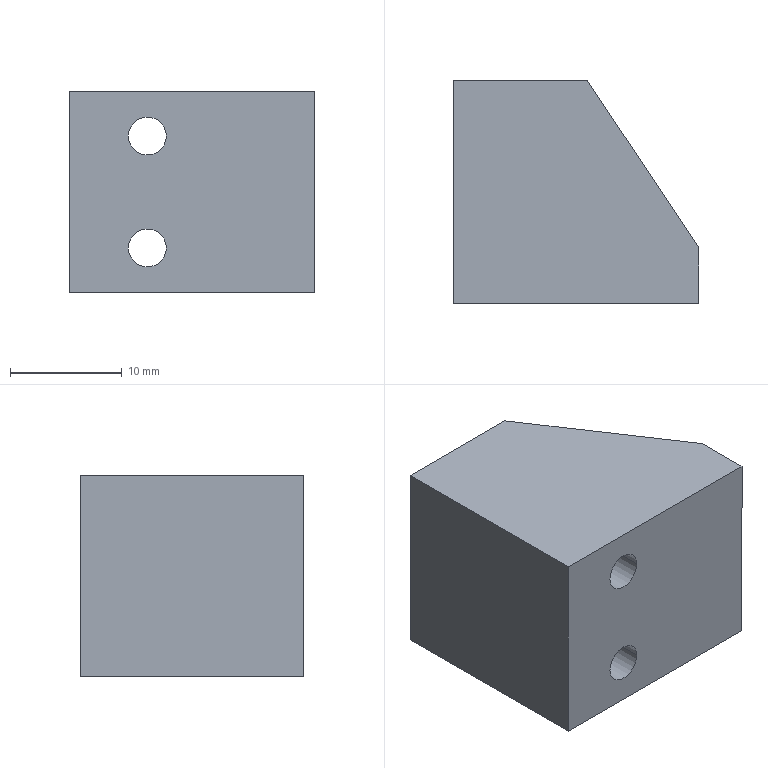Component | SolidWorks | XM-02-008A1-1 | 1 solid | 17 faces | box 22 x 20 x 18 mm | volume 5823 mm3 | plane 9 | cylinder 8 | commonest cylinder face diameters 6 x4 3.4 x4 | material Black POM
build123d program:
from build123d import *

# Parameters (mm, degrees)
SKETCH1_W                                          = 18
SKETCH1_H                                          = 22
BOSS_EXTRUDE1_DEPTH                                = 20
CUT_EXTRUDE1_DEPTH                                 = 20
HOLE_SIZE_ACCORDING_TO_TYPE_1_OF_HEX_S_D           = 3.4
HOLE_SIZE_ACCORDING_TO_TYPE_1_OF_HEX_S_CBORE_D     = 6
HOLE_SIZE_ACCORDING_TO_TYPE_1_OF_HEX_S_CBORE_DEPTH = 10


with BuildPart() as part:
    # Sketch1 → Boss-Extrude1 (new body)
    with BuildSketch(Plane(origin=(0, 0, 0), x_dir=(1, 0, 0), z_dir=(0, 1, 0))):
        Rectangle(SKETCH1_W, SKETCH1_H)
    extrude(amount=BOSS_EXTRUDE1_DEPTH)

    # Sketch14 → Cut-Extrude1 (cut)
    with BuildSketch(Plane.ZY.offset(9)):
        Polygon((-11, 20), (-1, 20), (-11, 5), align=None)
    extrude(amount=-CUT_EXTRUDE1_DEPTH, mode=Mode.SUBTRACT)

    # Hole Size _according to_ Type 1 of Hex S (through all)
    with Locations(Plane(origin=(0, 20, 0), x_dir=(1, 0, 0), z_dir=(0, 1, 0))):
        with Locations((5, -4), (-5, -4)):
            CounterBoreHole(HOLE_SIZE_ACCORDING_TO_TYPE_1_OF_HEX_S_D / 2, HOLE_SIZE_ACCORDING_TO_TYPE_1_OF_HEX_S_CBORE_D / 2, HOLE_SIZE_ACCORDING_TO_TYPE_1_OF_HEX_S_CBORE_DEPTH)


solid = part.part

# Placed as in the assembly
solid = solid.moved(Location((-54, 0, 0), (0, -90, 0)))
STEP:
#1=COLOUR_RGB('',0.7922,0.8196,0.9333);
#2=FILL_AREA_STYLE_COLOUR('',#1);
#3=FILL_AREA_STYLE('',(#2));
#4=SURFACE_STYLE_FILL_AREA(#3);
#5=SURFACE_SIDE_STYLE('',(#4));
#6=SURFACE_STYLE_USAGE(.BOTH.,#5);
#7=PRESENTATION_STYLE_ASSIGNMENT((#6));
#8=CARTESIAN_POINT('',(-2.165,0.3937,0.1969));
#9=VERTEX_POINT('',#8);
#10=CARTESIAN_POINT('',(-2.402,0.3937,0.1969));
#11=VERTEX_POINT('',#10);
#12=CARTESIAN_POINT('',(-2.283,0.3937,0.1969));
#13=DIRECTION('',(0.,1.,-0.));
#14=DIRECTION('',(-1.,0.,0.));
#15=AXIS2_PLACEMENT_3D('',#12,#13,#14);
#16=CIRCLE('',#15,0.1181);
#17=EDGE_CURVE('',#9,#11,#16,.T.);
#18=ORIENTED_EDGE('',*,*,#17,.F.);
#19=CARTESIAN_POINT('',(-2.165,0.7874,0.1969));
#20=VERTEX_POINT('',#19);
#21=CARTESIAN_POINT('',(-2.165,0.7874,0.1969));
#22=DIRECTION('',(0.,1.,-0.));
#23=VECTOR('',#22,39.37);
#24=LINE('',#21,#23);
#25=EDGE_CURVE('',#9,#20,#24,.T.);
#26=ORIENTED_EDGE('',*,*,#25,.T.);
#27=CARTESIAN_POINT('',(-2.402,0.7874,0.1969));
#28=VERTEX_POINT('',#27);
#29=CARTESIAN_POINT('',(-2.283,0.7874,0.1969));
#30=DIRECTION('',(0.,1.,-0.));
#31=DIRECTION('',(-1.,0.,0.));
#32=AXIS2_PLACEMENT_3D('',#29,#30,#31);
#33=CIRCLE('',#32,0.1181);
#34=EDGE_CURVE('',#20,#28,#33,.T.);
#35=ORIENTED_EDGE('',*,*,#34,.T.);
#36=CARTESIAN_POINT('',(-2.402,0.7874,0.1969));
#37=DIRECTION('',(0.,1.,-0.));
#38=VECTOR('',#37,39.37);
#39=LINE('',#36,#38);
#40=EDGE_CURVE('',#11,#28,#39,.T.);
#41=ORIENTED_EDGE('',*,*,#40,.F.);
#42=EDGE_LOOP('',(#18,#26,#35,#41));
#43=FACE_OUTER_BOUND('',#42,.T.);
#44=CARTESIAN_POINT('',(-2.283,0.7874,0.1969));
#45=DIRECTION('',(0.,1.,-0.));
#46=DIRECTION('',(-1.,0.,0.));
#47=AXIS2_PLACEMENT_3D('',#44,#45,#46);
#48=CYLINDRICAL_SURFACE('',#47,0.1181);
#49=ADVANCED_FACE('',(#43),#48,.F.);
#50=CARTESIAN_POINT('',(-2.217,0.,0.1969));
#51=VERTEX_POINT('',#50);
#52=CARTESIAN_POINT('',(-2.35,0.,0.1969));
#53=VERTEX_POINT('',#52);
#54=CARTESIAN_POINT('',(-2.283,0.,0.1969));
#55=DIRECTION('',(0.,1.,-0.));
#56=DIRECTION('',(-1.,0.,0.));
#57=AXIS2_PLACEMENT_3D('',#54,#55,#56);
#58=CIRCLE('',#57,0.06693);
#59=EDGE_CURVE('',#51,#53,#58,.T.);
#60=ORIENTED_EDGE('',*,*,#59,.F.);
#61=CARTESIAN_POINT('',(-2.217,0.3937,0.1969));
#62=VERTEX_POINT('',#61);
#63=CARTESIAN_POINT('',(-2.217,0.7874,0.1969));
#64=DIRECTION('',(0.,1.,-0.));
#65=VECTOR('',#64,39.37);
#66=LINE('',#63,#65);
#67=EDGE_CURVE('',#51,#62,#66,.T.);
#68=ORIENTED_EDGE('',*,*,#67,.T.);
#69=CARTESIAN_POINT('',(-2.35,0.3937,0.1969));
#70=VERTEX_POINT('',#69);
#71=CARTESIAN_POINT('',(-2.283,0.3937,0.1969));
#72=DIRECTION('',(0.,1.,-0.));
#73=DIRECTION('',(-1.,0.,0.));
#74=AXIS2_PLACEMENT_3D('',#71,#72,#73);
#75=CIRCLE('',#74,0.06693);
#76=EDGE_CURVE('',#62,#70,#75,.T.);
#77=ORIENTED_EDGE('',*,*,#76,.T.);
#78=CARTESIAN_POINT('',(-2.35,0.7874,0.1969));
#79=DIRECTION('',(0.,1.,-0.));
#80=VECTOR('',#79,39.37);
#81=LINE('',#78,#80);
#82=EDGE_CURVE('',#53,#70,#81,.T.);
#83=ORIENTED_EDGE('',*,*,#82,.F.);
#84=EDGE_LOOP('',(#60,#68,#77,#83));
#85=FACE_OUTER_BOUND('',#84,.T.);
#86=CARTESIAN_POINT('',(-2.283,0.7874,0.1969));
#87=DIRECTION('',(0.,1.,-0.));
#88=DIRECTION('',(-1.,0.,0.));
#89=AXIS2_PLACEMENT_3D('',#86,#87,#88);
#90=CYLINDRICAL_SURFACE('',#89,0.06693);
#91=ADVANCED_FACE('',(#85),#90,.F.);
#92=CARTESIAN_POINT('',(-2.165,0.3937,-0.1969));
#93=VERTEX_POINT('',#92);
#94=CARTESIAN_POINT('',(-2.402,0.3937,-0.1969));
#95=VERTEX_POINT('',#94);
#96=CARTESIAN_POINT('',(-2.283,0.3937,-0.1969));
#97=DIRECTION('',(0.,1.,-0.));
#98=DIRECTION('',(-1.,0.,0.));
#99=AXIS2_PLACEMENT_3D('',#96,#97,#98);
#100=CIRCLE('',#99,0.1181);
#101=EDGE_CURVE('',#93,#95,#100,.T.);
#102=ORIENTED_EDGE('',*,*,#101,.F.);
#103=CARTESIAN_POINT('',(-2.165,0.7874,-0.1969));
#104=VERTEX_POINT('',#103);
#105=CARTESIAN_POINT('',(-2.165,0.7874,-0.1969));
#106=DIRECTION('',(0.,1.,-0.));
#107=VECTOR('',#106,39.37);
#108=LINE('',#105,#107);
#109=EDGE_CURVE('',#93,#104,#108,.T.);
#110=ORIENTED_EDGE('',*,*,#109,.T.);
#111=CARTESIAN_POINT('',(-2.402,0.7874,-0.1969));
#112=VERTEX_POINT('',#111);
#113=CARTESIAN_POINT('',(-2.283,0.7874,-0.1969));
#114=DIRECTION('',(0.,1.,-0.));
#115=DIRECTION('',(-1.,0.,0.));
#116=AXIS2_PLACEMENT_3D('',#113,#114,#115);
#117=CIRCLE('',#116,0.1181);
#118=EDGE_CURVE('',#104,#112,#117,.T.);
#119=ORIENTED_EDGE('',*,*,#118,.T.);
#120=CARTESIAN_POINT('',(-2.402,0.7874,-0.1969));
#121=DIRECTION('',(0.,1.,-0.));
#122=VECTOR('',#121,39.37);
#123=LINE('',#120,#122);
#124=EDGE_CURVE('',#95,#112,#123,.T.);
#125=ORIENTED_EDGE('',*,*,#124,.F.);
#126=EDGE_LOOP('',(#102,#110,#119,#125));
#127=FACE_OUTER_BOUND('',#126,.T.);
#128=CARTESIAN_POINT('',(-2.283,0.7874,-0.1969));
#129=DIRECTION('',(0.,1.,-0.));
#130=DIRECTION('',(-1.,0.,0.));
#131=AXIS2_PLACEMENT_3D('',#128,#129,#130);
#132=CYLINDRICAL_SURFACE('',#131,0.1181);
#133=ADVANCED_FACE('',(#127),#132,.F.);
#134=CARTESIAN_POINT('',(-2.217,0.,-0.1969));
#135=VERTEX_POINT('',#134);
#136=CARTESIAN_POINT('',(-2.35,0.,-0.1969));
#137=VERTEX_POINT('',#136);
#138=CARTESIAN_POINT('',(-2.283,0.,-0.1969));
#139=DIRECTION('',(0.,1.,-0.));
#140=DIRECTION('',(-1.,0.,0.));
#141=AXIS2_PLACEMENT_3D('',#138,#139,#140);
#142=CIRCLE('',#141,0.06693);
#143=EDGE_CURVE('',#135,#137,#142,.T.);
#144=ORIENTED_EDGE('',*,*,#143,.F.);
#145=CARTESIAN_POINT('',(-2.217,0.3937,-0.1969));
#146=VERTEX_POINT('',#145);
#147=CARTESIAN_POINT('',(-2.217,0.7874,-0.1969));
#148=DIRECTION('',(0.,1.,-0.));
#149=VECTOR('',#148,39.37);
#150=LINE('',#147,#149);
#151=EDGE_CURVE('',#135,#146,#150,.T.);
#152=ORIENTED_EDGE('',*,*,#151,.T.);
#153=CARTESIAN_POINT('',(-2.35,0.3937,-0.1969));
#154=VERTEX_POINT('',#153);
#155=CARTESIAN_POINT('',(-2.283,0.3937,-0.1969));
#156=DIRECTION('',(0.,1.,-0.));
#157=DIRECTION('',(-1.,0.,0.));
#158=AXIS2_PLACEMENT_3D('',#155,#156,#157);
#159=CIRCLE('',#158,0.06693);
#160=EDGE_CURVE('',#146,#154,#159,.T.);
#161=ORIENTED_EDGE('',*,*,#160,.T.);
#162=CARTESIAN_POINT('',(-2.35,0.7874,-0.1969));
#163=DIRECTION('',(0.,1.,-0.));
#164=VECTOR('',#163,39.37);
#165=LINE('',#162,#164);
#166=EDGE_CURVE('',#137,#154,#165,.T.);
#167=ORIENTED_EDGE('',*,*,#166,.F.);
#168=EDGE_LOOP('',(#144,#152,#161,#167));
#169=FACE_OUTER_BOUND('',#168,.T.);
#170=CARTESIAN_POINT('',(-2.283,0.7874,-0.1969));
#171=DIRECTION('',(0.,1.,-0.));
#172=DIRECTION('',(-1.,0.,0.));
#173=AXIS2_PLACEMENT_3D('',#170,#171,#172);
#174=CYLINDRICAL_SURFACE('',#173,0.06693);
#175=ADVANCED_FACE('',(#169),#174,.F.);
#176=CARTESIAN_POINT('',(-1.693,0.1969,0.3543));
#177=VERTEX_POINT('',#176);
#178=CARTESIAN_POINT('',(-1.693,0.,0.3543));
#179=VERTEX_POINT('',#178);
#180=CARTESIAN_POINT('',(-1.693,0.7874,0.3543));
#181=DIRECTION('',(-0.,-1.,0.));
#182=VECTOR('',#181,39.37);
#183=LINE('',#180,#182);
#184=EDGE_CURVE('',#177,#179,#183,.T.);
#185=ORIENTED_EDGE('',*,*,#184,.F.);
#186=CARTESIAN_POINT('',(-2.087,0.7874,0.3543));
#187=VERTEX_POINT('',#186);
#188=CARTESIAN_POINT('',(-1.965,0.6057,0.3543));
#189=DIRECTION('',(-0.5547,0.8321,0.));
#190=VECTOR('',#189,39.37);
#191=LINE('',#188,#190);
#192=EDGE_CURVE('',#177,#187,#191,.T.);
#193=ORIENTED_EDGE('',*,*,#192,.T.);
#194=CARTESIAN_POINT('',(-2.559,0.7874,0.3543));
#195=VERTEX_POINT('',#194);
#196=CARTESIAN_POINT('',(-1.693,0.7874,0.3543));
#197=DIRECTION('',(1.,-0.,-0.));
#198=VECTOR('',#197,39.37);
#199=LINE('',#196,#198);
#200=EDGE_CURVE('',#195,#187,#199,.T.);
#201=ORIENTED_EDGE('',*,*,#200,.F.);
#202=CARTESIAN_POINT('',(-2.559,0.,0.3543));
#203=VERTEX_POINT('',#202);
#204=CARTESIAN_POINT('',(-2.559,0.7874,0.3543));
#205=DIRECTION('',(-0.,-1.,0.));
#206=VECTOR('',#205,39.37);
#207=LINE('',#204,#206);
#208=EDGE_CURVE('',#195,#203,#207,.T.);
#209=ORIENTED_EDGE('',*,*,#208,.T.);
#210=CARTESIAN_POINT('',(-1.693,0.,0.3543));
#211=DIRECTION('',(1.,-0.,-0.));
#212=VECTOR('',#211,39.37);
#213=LINE('',#210,#212);
#214=EDGE_CURVE('',#203,#179,#213,.T.);
#215=ORIENTED_EDGE('',*,*,#214,.T.);
#216=EDGE_LOOP('',(#185,#193,#201,#209,#215));
#217=FACE_OUTER_BOUND('',#216,.T.);
#218=CARTESIAN_POINT('',(-1.693,0.7874,0.3543));
#219=DIRECTION('',(-0.,-0.,-1.));
#220=DIRECTION('',(-1.,0.,0.));
#221=AXIS2_PLACEMENT_3D('',#218,#219,#220);
#222=PLANE('',#221);
#223=ADVANCED_FACE('',(#217),#222,.F.);
#224=CARTESIAN_POINT('',(-1.693,0.1969,-0.3543));
#225=VERTEX_POINT('',#224);
#226=CARTESIAN_POINT('',(-1.693,-0.,-0.3543));
#227=VERTEX_POINT('',#226);
#228=CARTESIAN_POINT('',(-1.693,0.7874,-0.3543));
#229=DIRECTION('',(-0.,-1.,0.));
#230=VECTOR('',#229,39.37);
#231=LINE('',#228,#230);
#232=EDGE_CURVE('',#225,#227,#231,.T.);
#233=ORIENTED_EDGE('',*,*,#232,.F.);
#234=CARTESIAN_POINT('',(-1.693,0.1969,0.4331));
#235=DIRECTION('',(-0.,-0.,-1.));
#236=VECTOR('',#235,39.37);
#237=LINE('',#234,#236);
#238=EDGE_CURVE('',#177,#225,#237,.T.);
#239=ORIENTED_EDGE('',*,*,#238,.F.);
#240=ORIENTED_EDGE('',*,*,#184,.T.);
#241=CARTESIAN_POINT('',(-1.693,-0.,-0.3543));
#242=DIRECTION('',(-0.,-0.,-1.));
#243=VECTOR('',#242,39.37);
#244=LINE('',#241,#243);
#245=EDGE_CURVE('',#179,#227,#244,.T.);
#246=ORIENTED_EDGE('',*,*,#245,.T.);
#247=EDGE_LOOP('',(#233,#239,#240,#246));
#248=FACE_OUTER_BOUND('',#247,.T.);
#249=CARTESIAN_POINT('',(-1.693,0.7874,-0.3543));
#250=DIRECTION('',(-1.,0.,0.));
#251=DIRECTION('',(0.,0.,1.));
#252=AXIS2_PLACEMENT_3D('',#249,#250,#251);
#253=PLANE('',#252);
#254=ADVANCED_FACE('',(#248),#253,.F.);
#255=CARTESIAN_POINT('',(-2.087,0.7874,-0.3543));
#256=VERTEX_POINT('',#255);
#257=CARTESIAN_POINT('',(-2.559,0.7874,-0.3543));
#258=VERTEX_POINT('',#257);
#259=CARTESIAN_POINT('',(-1.693,0.7874,-0.3543));
#260=DIRECTION('',(-1.,0.,0.));
#261=VECTOR('',#260,39.37);
#262=LINE('',#259,#261);
#263=EDGE_CURVE('',#256,#258,#262,.T.);
#264=ORIENTED_EDGE('',*,*,#263,.F.);
#265=CARTESIAN_POINT('',(-2.087,0.7874,-0.3543));
#266=DIRECTION('',(-0.5547,0.8321,0.));
#267=VECTOR('',#266,39.37);
#268=LINE('',#265,#267);
#269=EDGE_CURVE('',#225,#256,#268,.T.);
#270=ORIENTED_EDGE('',*,*,#269,.F.);
#271=ORIENTED_EDGE('',*,*,#232,.T.);
#272=CARTESIAN_POINT('',(-2.559,-0.,-0.3543));
#273=VERTEX_POINT('',#272);
#274=CARTESIAN_POINT('',(-1.693,-0.,-0.3543));
#275=DIRECTION('',(-1.,0.,0.));
#276=VECTOR('',#275,39.37);
#277=LINE('',#274,#276);
#278=EDGE_CURVE('',#227,#273,#277,.T.);
#279=ORIENTED_EDGE('',*,*,#278,.T.);
#280=CARTESIAN_POINT('',(-2.559,0.7874,-0.3543));
#281=DIRECTION('',(-0.,-1.,0.));
#282=VECTOR('',#281,39.37);
#283=LINE('',#280,#282);
#284=EDGE_CURVE('',#258,#273,#283,.T.);
#285=ORIENTED_EDGE('',*,*,#284,.F.);
#286=EDGE_LOOP('',(#264,#270,#271,#279,#285));
#287=FACE_OUTER_BOUND('',#286,.T.);
#288=CARTESIAN_POINT('',(-1.693,0.7874,-0.3543));
#289=DIRECTION('',(0.,0.,1.));
#290=DIRECTION('',(1.,-0.,-0.));
#291=AXIS2_PLACEMENT_3D('',#288,#289,#290);
#292=PLANE('',#291);
#293=ADVANCED_FACE('',(#287),#292,.F.);
#294=CARTESIAN_POINT('',(-2.559,-0.,-0.3543));
#295=DIRECTION('',(0.,0.,1.));
#296=VECTOR('',#295,39.37);
#297=LINE('',#294,#296);
#298=EDGE_CURVE('',#273,#203,#297,.T.);
#299=ORIENTED_EDGE('',*,*,#298,.T.);
#300=ORIENTED_EDGE('',*,*,#208,.F.);
#301=CARTESIAN_POINT('',(-2.559,0.7874,-0.3543));
#302=DIRECTION('',(0.,0.,1.));
#303=VECTOR('',#302,39.37);
#304=LINE('',#301,#303);
#305=EDGE_CURVE('',#258,#195,#304,.T.);
#306=ORIENTED_EDGE('',*,*,#305,.F.);
#307=ORIENTED_EDGE('',*,*,#284,.T.);
#308=EDGE_LOOP('',(#299,#300,#306,#307));
#309=FACE_OUTER_BOUND('',#308,.T.);
#310=CARTESIAN_POINT('',(-2.559,0.7874,-0.3543));
#311=DIRECTION('',(1.,-0.,-0.));
#312=DIRECTION('',(-0.,-0.,-1.));
#313=AXIS2_PLACEMENT_3D('',#310,#311,#312);
#314=PLANE('',#313);
#315=ADVANCED_FACE('',(#309),#314,.F.);
#316=CARTESIAN_POINT('',(-2.283,0.7874,0.1969));
#317=DIRECTION('',(0.,1.,-0.));
#318=DIRECTION('',(-1.,0.,0.));
#319=AXIS2_PLACEMENT_3D('',#316,#317,#318);
#320=CIRCLE('',#319,0.1181);
#321=EDGE_CURVE('',#28,#20,#320,.T.);
#322=ORIENTED_EDGE('',*,*,#321,.F.);
#323=ORIENTED_EDGE('',*,*,#34,.F.);
#324=EDGE_LOOP('',(#322,#323));
#325=FACE_BOUND('',#324,.T.);
#326=CARTESIAN_POINT('',(-2.283,0.7874,-0.1969));
#327=DIRECTION('',(0.,1.,-0.));
#328=DIRECTION('',(-1.,0.,0.));
#329=AXIS2_PLACEMENT_3D('',#326,#327,#328);
#330=CIRCLE('',#329,0.1181);
#331=EDGE_CURVE('',#112,#104,#330,.T.);
#332=ORIENTED_EDGE('',*,*,#331,.F.);
#333=ORIENTED_EDGE('',*,*,#118,.F.);
#334=EDGE_LOOP('',(#332,#333));
#335=FACE_BOUND('',#334,.T.);
#336=CARTESIAN_POINT('',(-2.087,0.7874,0.));
#337=DIRECTION('',(0.,0.,1.));
#338=VECTOR('',#337,39.37);
#339=LINE('',#336,#338);
#340=EDGE_CURVE('',#256,#187,#339,.T.);
#341=ORIENTED_EDGE('',*,*,#340,.F.);
#342=ORIENTED_EDGE('',*,*,#263,.T.);
#343=ORIENTED_EDGE('',*,*,#305,.T.);
#344=ORIENTED_EDGE('',*,*,#200,.T.);
#345=EDGE_LOOP('',(#341,#342,#343,#344));
#346=FACE_OUTER_BOUND('',#345,.T.);
#347=CARTESIAN_POINT('',(-2.126,0.7874,0.));
#348=DIRECTION('',(0.,1.,-0.));
#349=DIRECTION('',(-1.,0.,0.));
#350=AXIS2_PLACEMENT_3D('',#347,#348,#349);
#351=PLANE('',#350);
#352=ADVANCED_FACE('',(#325,#335,#346),#351,.T.);
#353=CARTESIAN_POINT('',(-2.283,0.,0.1969));
#354=DIRECTION('',(0.,1.,-0.));
#355=DIRECTION('',(-1.,0.,0.));
#356=AXIS2_PLACEMENT_3D('',#353,#354,#355);
#357=CIRCLE('',#356,0.06693);
#358=EDGE_CURVE('',#53,#51,#357,.T.);
#359=ORIENTED_EDGE('',*,*,#358,.T.);
#360=ORIENTED_EDGE('',*,*,#59,.T.);
#361=EDGE_LOOP('',(#359,#360));
#362=FACE_BOUND('',#361,.T.);
#363=CARTESIAN_POINT('',(-2.283,0.,-0.1969));
#364=DIRECTION('',(0.,1.,-0.));
#365=DIRECTION('',(-1.,0.,0.));
#366=AXIS2_PLACEMENT_3D('',#363,#364,#365);
#367=CIRCLE('',#366,0.06693);
#368=EDGE_CURVE('',#137,#135,#367,.T.);
#369=ORIENTED_EDGE('',*,*,#368,.T.);
#370=ORIENTED_EDGE('',*,*,#143,.T.);
#371=EDGE_LOOP('',(#369,#370));
#372=FACE_BOUND('',#371,.T.);
#373=ORIENTED_EDGE('',*,*,#214,.F.);
#374=ORIENTED_EDGE('',*,*,#298,.F.);
#375=ORIENTED_EDGE('',*,*,#278,.F.);
#376=ORIENTED_EDGE('',*,*,#245,.F.);
#377=EDGE_LOOP('',(#373,#374,#375,#376));
#378=FACE_OUTER_BOUND('',#377,.T.);
#379=CARTESIAN_POINT('',(-2.126,0.,0.));
#380=DIRECTION('',(0.,1.,-0.));
#381=DIRECTION('',(-1.,0.,0.));
#382=AXIS2_PLACEMENT_3D('',#379,#380,#381);
#383=PLANE('',#382);
#384=ADVANCED_FACE('',(#362,#372,#378),#383,.F.);
#385=ORIENTED_EDGE('',*,*,#238,.T.);
#386=ORIENTED_EDGE('',*,*,#269,.T.);
#387=ORIENTED_EDGE('',*,*,#340,.T.);
#388=ORIENTED_EDGE('',*,*,#192,.F.);
#389=EDGE_LOOP('',(#385,#386,#387,#388));
#390=FACE_OUTER_BOUND('',#389,.T.);
#391=CARTESIAN_POINT('',(-2.087,0.7874,0.4331));
#392=DIRECTION('',(-0.8321,-0.5547,0.));
#393=DIRECTION('',(0.5547,-0.8321,-0.));
#394=AXIS2_PLACEMENT_3D('',#391,#392,#393);
#395=PLANE('',#394);
#396=ADVANCED_FACE('',(#390),#395,.F.);
#397=ORIENTED_EDGE('',*,*,#151,.F.);
#398=ORIENTED_EDGE('',*,*,#368,.F.);
#399=ORIENTED_EDGE('',*,*,#166,.T.);
#400=CARTESIAN_POINT('',(-2.283,0.3937,-0.1969));
#401=DIRECTION('',(0.,1.,-0.));
#402=DIRECTION('',(-1.,0.,0.));
#403=AXIS2_PLACEMENT_3D('',#400,#401,#402);
#404=CIRCLE('',#403,0.06693);
#405=EDGE_CURVE('',#154,#146,#404,.T.);
#406=ORIENTED_EDGE('',*,*,#405,.T.);
#407=EDGE_LOOP('',(#397,#398,#399,#406));
#408=FACE_OUTER_BOUND('',#407,.T.);
#409=CARTESIAN_POINT('',(-2.283,0.7874,-0.1969));
#410=DIRECTION('',(0.,1.,-0.));
#411=DIRECTION('',(-1.,0.,0.));
#412=AXIS2_PLACEMENT_3D('',#409,#410,#411);
#413=CYLINDRICAL_SURFACE('',#412,0.06693);
#414=ADVANCED_FACE('',(#408),#413,.F.);
#415=ORIENTED_EDGE('',*,*,#405,.F.);
#416=ORIENTED_EDGE('',*,*,#160,.F.);
#417=EDGE_LOOP('',(#415,#416));
#418=FACE_BOUND('',#417,.T.);
#419=CARTESIAN_POINT('',(-2.283,0.3937,-0.1969));
#420=DIRECTION('',(0.,1.,-0.));
#421=DIRECTION('',(-1.,0.,0.));
#422=AXIS2_PLACEMENT_3D('',#419,#420,#421);
#423=CIRCLE('',#422,0.1181);
#424=EDGE_CURVE('',#95,#93,#423,.T.);
#425=ORIENTED_EDGE('',*,*,#424,.T.);
#426=ORIENTED_EDGE('',*,*,#101,.T.);
#427=EDGE_LOOP('',(#425,#426));
#428=FACE_OUTER_BOUND('',#427,.T.);
#429=CARTESIAN_POINT('',(-2.283,0.3937,-0.1299));
#430=DIRECTION('',(-0.,-1.,0.));
#431=DIRECTION('',(1.,-0.,-0.));
#432=AXIS2_PLACEMENT_3D('',#429,#430,#431);
#433=PLANE('',#432);
#434=ADVANCED_FACE('',(#418,#428),#433,.F.);
#435=ORIENTED_EDGE('',*,*,#109,.F.);
#436=ORIENTED_EDGE('',*,*,#424,.F.);
#437=ORIENTED_EDGE('',*,*,#124,.T.);
#438=ORIENTED_EDGE('',*,*,#331,.T.);
#439=EDGE_LOOP('',(#435,#436,#437,#438));
#440=FACE_OUTER_BOUND('',#439,.T.);
#441=CARTESIAN_POINT('',(-2.283,0.7874,-0.1969));
#442=DIRECTION('',(0.,1.,-0.));
#443=DIRECTION('',(-1.,0.,0.));
#444=AXIS2_PLACEMENT_3D('',#441,#442,#443);
#445=CYLINDRICAL_SURFACE('',#444,0.1181);
#446=ADVANCED_FACE('',(#440),#445,.F.);
#447=ORIENTED_EDGE('',*,*,#67,.F.);
#448=ORIENTED_EDGE('',*,*,#358,.F.);
#449=ORIENTED_EDGE('',*,*,#82,.T.);
#450=CARTESIAN_POINT('',(-2.283,0.3937,0.1969));
#451=DIRECTION('',(0.,1.,-0.));
#452=DIRECTION('',(-1.,0.,0.));
#453=AXIS2_PLACEMENT_3D('',#450,#451,#452);
#454=CIRCLE('',#453,0.06693);
#455=EDGE_CURVE('',#70,#62,#454,.T.);
#456=ORIENTED_EDGE('',*,*,#455,.T.);
#457=EDGE_LOOP('',(#447,#448,#449,#456));
#458=FACE_OUTER_BOUND('',#457,.T.);
#459=CARTESIAN_POINT('',(-2.283,0.7874,0.1969));
#460=DIRECTION('',(0.,1.,-0.));
#461=DIRECTION('',(-1.,0.,0.));
#462=AXIS2_PLACEMENT_3D('',#459,#460,#461);
#463=CYLINDRICAL_SURFACE('',#462,0.06693);
#464=ADVANCED_FACE('',(#458),#463,.F.);
#465=ORIENTED_EDGE('',*,*,#455,.F.);
#466=ORIENTED_EDGE('',*,*,#76,.F.);
#467=EDGE_LOOP('',(#465,#466));
#468=FACE_BOUND('',#467,.T.);
#469=CARTESIAN_POINT('',(-2.283,0.3937,0.1969));
#470=DIRECTION('',(0.,1.,-0.));
#471=DIRECTION('',(-1.,0.,0.));
#472=AXIS2_PLACEMENT_3D('',#469,#470,#471);
#473=CIRCLE('',#472,0.1181);
#474=EDGE_CURVE('',#11,#9,#473,.T.);
#475=ORIENTED_EDGE('',*,*,#474,.T.);
#476=ORIENTED_EDGE('',*,*,#17,.T.);
#477=EDGE_LOOP('',(#475,#476));
#478=FACE_OUTER_BOUND('',#477,.T.);
#479=CARTESIAN_POINT('',(-2.283,0.3937,0.2638));
#480=DIRECTION('',(-0.,-1.,0.));
#481=DIRECTION('',(1.,-0.,-0.));
#482=AXIS2_PLACEMENT_3D('',#479,#480,#481);
#483=PLANE('',#482);
#484=ADVANCED_FACE('',(#468,#478),#483,.F.);
#485=ORIENTED_EDGE('',*,*,#25,.F.);
#486=ORIENTED_EDGE('',*,*,#474,.F.);
#487=ORIENTED_EDGE('',*,*,#40,.T.);
#488=ORIENTED_EDGE('',*,*,#321,.T.);
#489=EDGE_LOOP('',(#485,#486,#487,#488));
#490=FACE_OUTER_BOUND('',#489,.T.);
#491=CARTESIAN_POINT('',(-2.283,0.7874,0.1969));
#492=DIRECTION('',(0.,1.,-0.));
#493=DIRECTION('',(-1.,0.,0.));
#494=AXIS2_PLACEMENT_3D('',#491,#492,#493);
#495=CYLINDRICAL_SURFACE('',#494,0.1181);
#496=ADVANCED_FACE('',(#490),#495,.F.);
#497=CLOSED_SHELL('',(#49,#91,#133,#175,#223,#254,#293,#315,#352,#384,#396,#414,#434,#446,#464,#484,#496));
#498=MANIFOLD_SOLID_BREP('',#497);
#499=STYLED_ITEM('',(#7),#498);
#500=(LENGTH_UNIT()NAMED_UNIT(*)SI_UNIT($,.METRE.));
#501=LENGTH_MEASURE_WITH_UNIT(LENGTH_MEASURE(0.0254),#500);
#502=DIMENSIONAL_EXPONENTS(1.,0.,0.,0.,0.,0.,0.);
#503=(CONVERSION_BASED_UNIT('',#501)LENGTH_UNIT()NAMED_UNIT(#502));
#504=UNCERTAINTY_MEASURE_WITH_UNIT(LENGTH_MEASURE(0.00001),#503,'','');
#505=(NAMED_UNIT(*)PLANE_ANGLE_UNIT()SI_UNIT($,.RADIAN.));
#506=(NAMED_UNIT(*)SI_UNIT($,.STERADIAN.)SOLID_ANGLE_UNIT());
#507=(GEOMETRIC_REPRESENTATION_CONTEXT(3)GLOBAL_UNCERTAINTY_ASSIGNED_CONTEXT((#504))GLOBAL_UNIT_ASSIGNED_CONTEXT((#503,#505,#506))REPRESENTATION_CONTEXT('',''));
#508=MECHANICAL_DESIGN_GEOMETRIC_PRESENTATION_REPRESENTATION('',(#499),#507);
#509=CARTESIAN_POINT('',(0.,0.,0.));
#510=DIRECTION('',(0.,0.,1.));
#511=DIRECTION('',(1.,0.,0.));
#512=AXIS2_PLACEMENT_3D('',#509,#510,#511);
#513=(LENGTH_UNIT()NAMED_UNIT(*)SI_UNIT($,.METRE.));
#514=LENGTH_MEASURE_WITH_UNIT(LENGTH_MEASURE(0.0254),#513);
#515=DIMENSIONAL_EXPONENTS(1.,0.,0.,0.,0.,0.,0.);
#516=(CONVERSION_BASED_UNIT('',#514)LENGTH_UNIT()NAMED_UNIT(#515));
#517=UNCERTAINTY_MEASURE_WITH_UNIT(LENGTH_MEASURE(0.00001),#516,'','');
#518=(NAMED_UNIT(*)PLANE_ANGLE_UNIT()SI_UNIT($,.RADIAN.));
#519=(NAMED_UNIT(*)SI_UNIT($,.STERADIAN.)SOLID_ANGLE_UNIT());
#520=(GEOMETRIC_REPRESENTATION_CONTEXT(3)GLOBAL_UNCERTAINTY_ASSIGNED_CONTEXT((#517))GLOBAL_UNIT_ASSIGNED_CONTEXT((#516,#518,#519))REPRESENTATION_CONTEXT('',''));
#521=ADVANCED_BREP_SHAPE_REPRESENTATION('',(#498,#512),#520);
#522=PRESENTATION_LAYER_ASSIGNMENT('','',(#499));